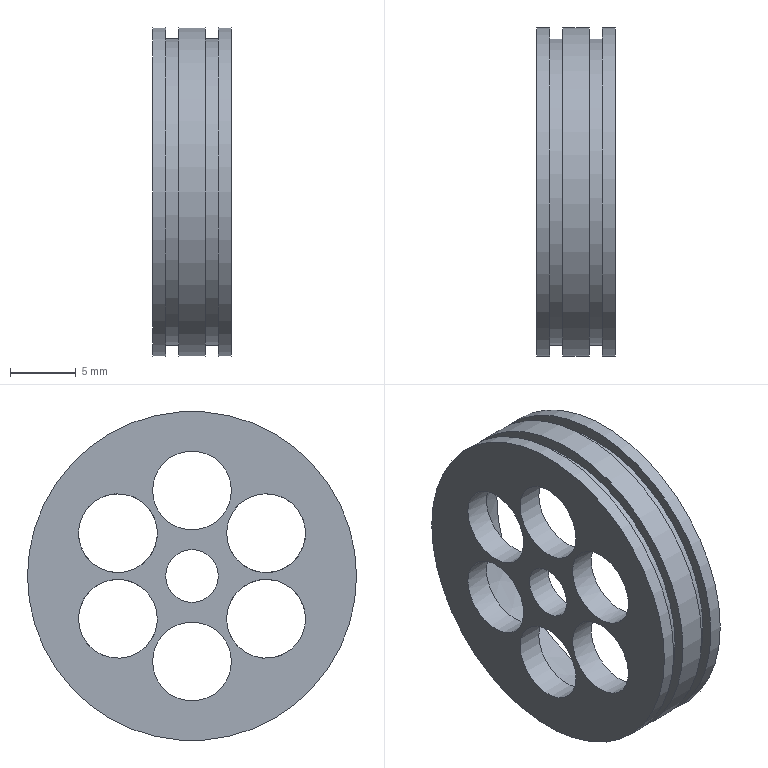Component | NX | INT_PIPE_FLYWHEEL | 1 solid | 20 faces | volume 997 mm3 | cylinder 12 | plane 7 | cone 1 | commonest cylinder face diameters 6 x6 25 x3 23.3 x2 4 x1